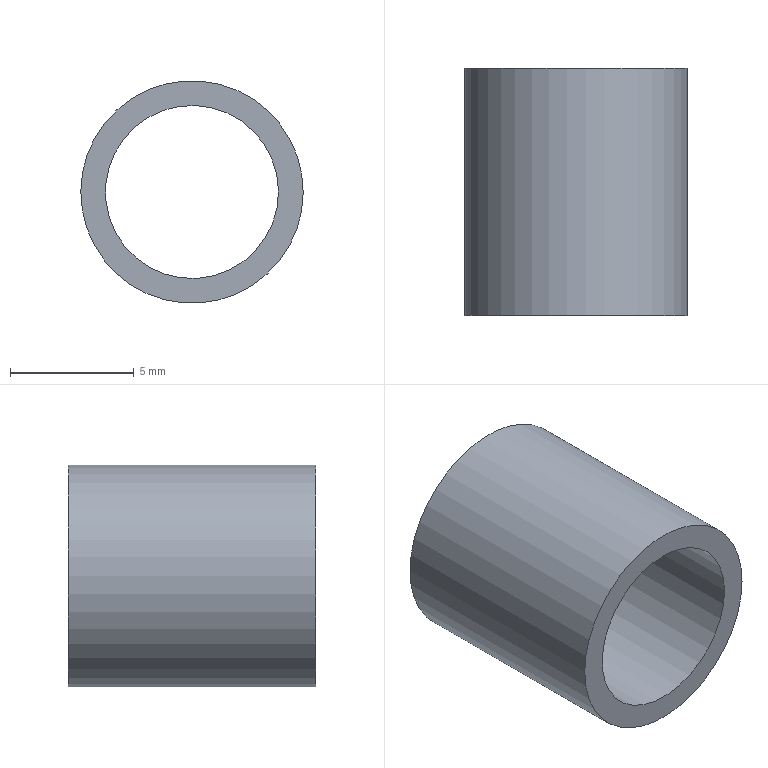Component | NX | BOTTOM_BEARING_SHELL | 1 solid | 4 faces | volume 251 mm3 | cylinder 2 | plane 2 | commonest cylinder face diameters 9 x1 7 x1